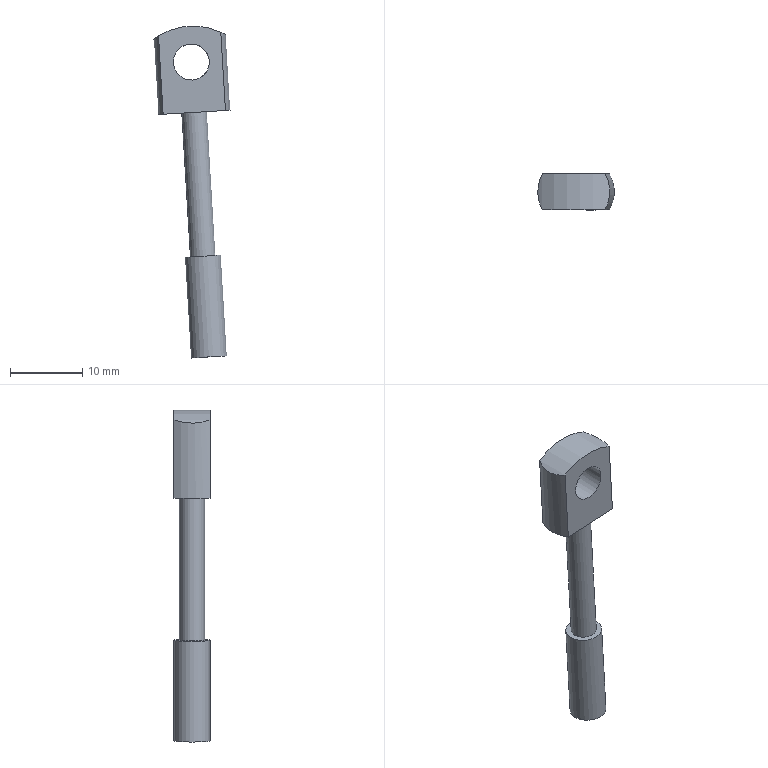Component | NX | PISTON_CONN_ROD | 1 solid | 11 faces | box 10.61 x 5 x 46.08 mm | volume 922 mm3 | cylinder 6 | plane 5 | commonest cylinder face diameters 5 x2 10 x2 18 x1 3.5 x1
STEP:
#1=CARTESIAN_POINT('',(0.,0.,0.));
#2=DIRECTION('',(0.,0.,1.));
#3=DIRECTION('',(1.,0.,0.));
#4=AXIS2_PLACEMENT_3D('',#1,#2,#3);
#5=CARTESIAN_POINT('',(4.091,25.5,90.772));
#6=VERTEX_POINT('',#5);
#7=CARTESIAN_POINT('',(4.091,20.5,90.772));
#8=VERTEX_POINT('',#7);
#9=CARTESIAN_POINT('',(4.091,25.5,90.772));
#10=CARTESIAN_POINT('',(4.534,24.755,90.562));
#11=CARTESIAN_POINT('',(4.784,23.892,90.406));
#12=CARTESIAN_POINT('',(4.783,22.106,90.406));
#13=CARTESIAN_POINT('',(4.534,21.245,90.562));
#14=CARTESIAN_POINT('',(4.091,20.5,90.772));
#15=B_SPLINE_CURVE_WITH_KNOTS('',3,(#9,#10,#11,#12,#13,#14),.UNSPECIFIED.,.F.,.F.,(4,2,4),(0.,0.5,1.),.UNSPECIFIED.);
#16=CARTESIAN_POINT('',(0.2383,20.5,82.638));
#17=DIRECTION('',(0.,1.,0.));
#18=DIRECTION('',(-0.05959,0.,0.9982));
#19=AXIS2_PLACEMENT_3D('',#16,#17,#18);
#20=CYLINDRICAL_SURFACE('',#19,9.);
#21=CARTESIAN_POINT('',(0.5019,5.));
#22=CARTESIAN_POINT('',(0.5069,4.932));
#23=CARTESIAN_POINT('',(0.5164,4.795));
#24=CARTESIAN_POINT('',(0.5296,4.583));
#25=CARTESIAN_POINT('',(0.5416,4.367));
#26=CARTESIAN_POINT('',(0.5524,4.146));
#27=CARTESIAN_POINT('',(0.5619,3.92));
#28=CARTESIAN_POINT('',(0.5701,3.691));
#29=CARTESIAN_POINT('',(0.5768,3.458));
#30=CARTESIAN_POINT('',(0.5822,3.222));
#31=CARTESIAN_POINT('',(0.5861,2.983));
#32=CARTESIAN_POINT('',(0.5885,2.742));
#33=CARTESIAN_POINT('',(0.5893,2.499));
#34=CARTESIAN_POINT('',(0.5885,2.256));
#35=CARTESIAN_POINT('',(0.5861,2.015));
#36=CARTESIAN_POINT('',(0.5822,1.777));
#37=CARTESIAN_POINT('',(0.5768,1.541));
#38=CARTESIAN_POINT('',(0.57,1.308));
#39=CARTESIAN_POINT('',(0.5619,1.079));
#40=CARTESIAN_POINT('',(0.5524,0.8538));
#41=CARTESIAN_POINT('',(0.5416,0.6329));
#42=CARTESIAN_POINT('',(0.5296,0.4165));
#43=CARTESIAN_POINT('',(0.5164,0.2051));
#44=CARTESIAN_POINT('',(0.5069,0.06772));
#45=CARTESIAN_POINT('',(0.5019,0.));
#46=B_SPLINE_CURVE_WITH_KNOTS('',3,(#21,#22,#23,#24,#25,#26,#27,#28,#29,#30,#31,#32,#33,#34,#35,#36,#37,#38,#39,#40,#41,#42,#43,#44,#45),.UNSPECIFIED.,.F.,.F.,(4,1,1,1,1,1,1,1,1,1,1,1,1,1,1,1,1,1,1,1,1,1,4),(0.,0.04545,0.09091,0.1364,0.1818,0.2273,0.2727,0.3182,0.3636,0.4091,0.4545,0.5,0.5455,0.5909,0.6364,0.6818,0.7273,0.7727,0.8182,0.8636,0.9091,0.9545,1.),.QUASI_UNIFORM_KNOTS.);
#47=(GEOMETRIC_REPRESENTATION_CONTEXT(2)PARAMETRIC_REPRESENTATION_CONTEXT()REPRESENTATION_CONTEXT('',''));
#48=DEFINITIONAL_REPRESENTATION('',(#46),#47);
#49=PCURVE('',#20,#48);
#50=CARTESIAN_POINT('',(-0.5363,23.,95.615));
#51=DIRECTION('',(0.05959,0.,-0.9982));
#52=DIRECTION('',(0.,1.,0.));
#53=AXIS2_PLACEMENT_3D('',#50,#51,#52);
#54=CYLINDRICAL_SURFACE('',#53,5.);
#55=CARTESIAN_POINT('',(1.047,5.11));
#56=CARTESIAN_POINT('',(1.063,5.132));
#57=CARTESIAN_POINT('',(1.094,5.173));
#58=CARTESIAN_POINT('',(1.141,5.232));
#59=CARTESIAN_POINT('',(1.188,5.287));
#60=CARTESIAN_POINT('',(1.236,5.337));
#61=CARTESIAN_POINT('',(1.283,5.382));
#62=CARTESIAN_POINT('',(1.33,5.422));
#63=CARTESIAN_POINT('',(1.378,5.455));
#64=CARTESIAN_POINT('',(1.426,5.482));
#65=CARTESIAN_POINT('',(1.474,5.502));
#66=CARTESIAN_POINT('',(1.522,5.514));
#67=CARTESIAN_POINT('',(1.571,5.518));
#68=CARTESIAN_POINT('',(1.62,5.514));
#69=CARTESIAN_POINT('',(1.668,5.502));
#70=CARTESIAN_POINT('',(1.716,5.482));
#71=CARTESIAN_POINT('',(1.764,5.455));
#72=CARTESIAN_POINT('',(1.811,5.422));
#73=CARTESIAN_POINT('',(1.859,5.382));
#74=CARTESIAN_POINT('',(1.906,5.337));
#75=CARTESIAN_POINT('',(1.953,5.287));
#76=CARTESIAN_POINT('',(2.,5.232));
#77=CARTESIAN_POINT('',(2.047,5.173));
#78=CARTESIAN_POINT('',(2.079,5.132));
#79=CARTESIAN_POINT('',(2.094,5.11));
#80=B_SPLINE_CURVE_WITH_KNOTS('',3,(#55,#56,#57,#58,#59,#60,#61,#62,#63,#64,#65,#66,#67,#68,#69,#70,#71,#72,#73,#74,#75,#76,#77,#78,#79),.UNSPECIFIED.,.F.,.F.,(4,1,1,1,1,1,1,1,1,1,1,1,1,1,1,1,1,1,1,1,1,1,4),(0.,0.04545,0.09091,0.1364,0.1818,0.2273,0.2727,0.3182,0.3636,0.4091,0.4545,0.5,0.5455,0.5909,0.6364,0.6818,0.7273,0.7727,0.8182,0.8636,0.9091,0.9545,1.),.QUASI_UNIFORM_KNOTS.);
#81=(GEOMETRIC_REPRESENTATION_CONTEXT(2)PARAMETRIC_REPRESENTATION_CONTEXT()REPRESENTATION_CONTEXT('',''));
#82=DEFINITIONAL_REPRESENTATION('',(#80),#81);
#83=PCURVE('',#54,#82);
#84=SURFACE_CURVE('',#15,(#49,#83),.PCURVE_S1.);
#85=EDGE_CURVE('',#6,#8,#84,.T.);
#86=ORIENTED_EDGE('',*,*,#85,.F.);
#87=CARTESIAN_POINT('',(-4.554,25.5,90.256));
#88=VERTEX_POINT('',#87);
#89=CARTESIAN_POINT('',(0.2383,25.5,82.638));
#90=DIRECTION('',(0.,-1.,0.));
#91=DIRECTION('',(0.9982,0.,0.05959));
#92=AXIS2_PLACEMENT_3D('',#89,#90,#91);
#93=CIRCLE('',#92,9.);
#94=CARTESIAN_POINT('',(1.571,5.));
#95=DIRECTION('',(-1.,0.));
#96=VECTOR('',#95,1.);
#97=LINE('',#94,#96);
#98=(GEOMETRIC_REPRESENTATION_CONTEXT(2)PARAMETRIC_REPRESENTATION_CONTEXT()REPRESENTATION_CONTEXT('',''));
#99=DEFINITIONAL_REPRESENTATION('',(#97),#98);
#100=PCURVE('',#20,#99);
#101=CARTESIAN_POINT('',(0.2383,25.5,82.638));
#102=DIRECTION('',(0.,-1.,0.));
#103=DIRECTION('',(0.05959,0.,-0.9982));
#104=AXIS2_PLACEMENT_3D('',#101,#102,#103);
#105=PLANE('',#104);
#106=CARTESIAN_POINT('',(0.,0.));
#107=DIRECTION('',(-0.,1.));
#108=AXIS2_PLACEMENT_2D('',#106,#107);
#109=CIRCLE('',#108,9.);
#110=(GEOMETRIC_REPRESENTATION_CONTEXT(2)PARAMETRIC_REPRESENTATION_CONTEXT()REPRESENTATION_CONTEXT('',''));
#111=DEFINITIONAL_REPRESENTATION('',(#109),#110);
#112=PCURVE('',#105,#111);
#113=SURFACE_CURVE('',#93,(#100,#112),.PCURVE_S1.);
#114=EDGE_CURVE('',#6,#88,#113,.T.);
#115=ORIENTED_EDGE('',*,*,#114,.T.);
#116=CARTESIAN_POINT('',(-4.554,20.5,90.256));
#117=VERTEX_POINT('',#116);
#118=CARTESIAN_POINT('',(-4.554,25.5,90.256));
#119=CARTESIAN_POINT('',(-4.969,24.755,89.994));
#120=CARTESIAN_POINT('',(-5.199,23.892,89.81));
#121=CARTESIAN_POINT('',(-5.198,22.106,89.81));
#122=CARTESIAN_POINT('',(-4.969,21.245,89.994));
#123=CARTESIAN_POINT('',(-4.554,20.5,90.256));
#124=B_SPLINE_CURVE_WITH_KNOTS('',3,(#118,#119,#120,#121,#122,#123),.UNSPECIFIED.,.F.,.F.,(4,2,4),(0.,0.5,1.),.UNSPECIFIED.);
#125=CARTESIAN_POINT('',(-0.5019,5.));
#126=CARTESIAN_POINT('',(-0.5069,4.932));
#127=CARTESIAN_POINT('',(-0.5164,4.795));
#128=CARTESIAN_POINT('',(-0.5296,4.583));
#129=CARTESIAN_POINT('',(-0.5416,4.367));
#130=CARTESIAN_POINT('',(-0.5524,4.146));
#131=CARTESIAN_POINT('',(-0.5619,3.92));
#132=CARTESIAN_POINT('',(-0.5701,3.691));
#133=CARTESIAN_POINT('',(-0.5768,3.458));
#134=CARTESIAN_POINT('',(-0.5822,3.222));
#135=CARTESIAN_POINT('',(-0.5861,2.983));
#136=CARTESIAN_POINT('',(-0.5885,2.742));
#137=CARTESIAN_POINT('',(-0.5893,2.499));
#138=CARTESIAN_POINT('',(-0.5885,2.256));
#139=CARTESIAN_POINT('',(-0.5861,2.015));
#140=CARTESIAN_POINT('',(-0.5822,1.777));
#141=CARTESIAN_POINT('',(-0.5768,1.541));
#142=CARTESIAN_POINT('',(-0.57,1.308));
#143=CARTESIAN_POINT('',(-0.5619,1.079));
#144=CARTESIAN_POINT('',(-0.5524,0.8538));
#145=CARTESIAN_POINT('',(-0.5416,0.6329));
#146=CARTESIAN_POINT('',(-0.5296,0.4165));
#147=CARTESIAN_POINT('',(-0.5164,0.2051));
#148=CARTESIAN_POINT('',(-0.5069,0.06772));
#149=CARTESIAN_POINT('',(-0.5019,0.));
#150=B_SPLINE_CURVE_WITH_KNOTS('',3,(#125,#126,#127,#128,#129,#130,#131,#132,#133,#134,#135,#136,#137,#138,#139,#140,#141,#142,#143,#144,#145,#146,#147,#148,#149),.UNSPECIFIED.,.F.,.F.,(4,1,1,1,1,1,1,1,1,1,1,1,1,1,1,1,1,1,1,1,1,1,4),(0.,0.04545,0.09091,0.1364,0.1818,0.2273,0.2727,0.3182,0.3636,0.4091,0.4545,0.5,0.5455,0.5909,0.6364,0.6818,0.7273,0.7727,0.8182,0.8636,0.9091,0.9545,1.),.QUASI_UNIFORM_KNOTS.);
#151=(GEOMETRIC_REPRESENTATION_CONTEXT(2)PARAMETRIC_REPRESENTATION_CONTEXT()REPRESENTATION_CONTEXT('',''));
#152=DEFINITIONAL_REPRESENTATION('',(#150),#151);
#153=PCURVE('',#20,#152);
#154=CARTESIAN_POINT('',(-0.5363,23.,95.615));
#155=DIRECTION('',(0.05959,0.,-0.9982));
#156=DIRECTION('',(0.,1.,0.));
#157=AXIS2_PLACEMENT_3D('',#154,#155,#156);
#158=CYLINDRICAL_SURFACE('',#157,5.);
#159=CARTESIAN_POINT('',(5.236,5.11));
#160=CARTESIAN_POINT('',(5.22,5.132));
#161=CARTESIAN_POINT('',(5.189,5.173));
#162=CARTESIAN_POINT('',(5.142,5.232));
#163=CARTESIAN_POINT('',(5.095,5.287));
#164=CARTESIAN_POINT('',(5.048,5.337));
#165=CARTESIAN_POINT('',(5.,5.382));
#166=CARTESIAN_POINT('',(4.953,5.422));
#167=CARTESIAN_POINT('',(4.905,5.455));
#168=CARTESIAN_POINT('',(4.857,5.482));
#169=CARTESIAN_POINT('',(4.809,5.502));
#170=CARTESIAN_POINT('',(4.761,5.514));
#171=CARTESIAN_POINT('',(4.712,5.518));
#172=CARTESIAN_POINT('',(4.664,5.514));
#173=CARTESIAN_POINT('',(4.615,5.502));
#174=CARTESIAN_POINT('',(4.567,5.482));
#175=CARTESIAN_POINT('',(4.519,5.455));
#176=CARTESIAN_POINT('',(4.472,5.422));
#177=CARTESIAN_POINT('',(4.424,5.382));
#178=CARTESIAN_POINT('',(4.377,5.337));
#179=CARTESIAN_POINT('',(4.33,5.287));
#180=CARTESIAN_POINT('',(4.283,5.232));
#181=CARTESIAN_POINT('',(4.236,5.173));
#182=CARTESIAN_POINT('',(4.204,5.132));
#183=CARTESIAN_POINT('',(4.189,5.11));
#184=B_SPLINE_CURVE_WITH_KNOTS('',3,(#159,#160,#161,#162,#163,#164,#165,#166,#167,#168,#169,#170,#171,#172,#173,#174,#175,#176,#177,#178,#179,#180,#181,#182,#183),.UNSPECIFIED.,.F.,.F.,(4,1,1,1,1,1,1,1,1,1,1,1,1,1,1,1,1,1,1,1,1,1,4),(0.,0.04545,0.09091,0.1364,0.1818,0.2273,0.2727,0.3182,0.3636,0.4091,0.4545,0.5,0.5455,0.5909,0.6364,0.6818,0.7273,0.7727,0.8182,0.8636,0.9091,0.9545,1.),.QUASI_UNIFORM_KNOTS.);
#185=(GEOMETRIC_REPRESENTATION_CONTEXT(2)PARAMETRIC_REPRESENTATION_CONTEXT()REPRESENTATION_CONTEXT('',''));
#186=DEFINITIONAL_REPRESENTATION('',(#184),#185);
#187=PCURVE('',#158,#186);
#188=SURFACE_CURVE('',#124,(#153,#187),.PCURVE_S1.);
#189=EDGE_CURVE('',#88,#117,#188,.T.);
#190=ORIENTED_EDGE('',*,*,#189,.T.);
#191=CARTESIAN_POINT('',(0.2383,20.5,82.638));
#192=DIRECTION('',(0.,-1.,0.));
#193=DIRECTION('',(0.9982,0.,0.05959));
#194=AXIS2_PLACEMENT_3D('',#191,#192,#193);
#195=CIRCLE('',#194,9.);
#196=CARTESIAN_POINT('',(1.571,0.));
#197=DIRECTION('',(-1.,0.));
#198=VECTOR('',#197,1.);
#199=LINE('',#196,#198);
#200=(GEOMETRIC_REPRESENTATION_CONTEXT(2)PARAMETRIC_REPRESENTATION_CONTEXT()REPRESENTATION_CONTEXT('',''));
#201=DEFINITIONAL_REPRESENTATION('',(#199),#200);
#202=PCURVE('',#20,#201);
#203=CARTESIAN_POINT('',(0.2383,20.5,82.638));
#204=DIRECTION('',(0.,-1.,0.));
#205=DIRECTION('',(0.05959,0.,-0.9982));
#206=AXIS2_PLACEMENT_3D('',#203,#204,#205);
#207=PLANE('',#206);
#208=CARTESIAN_POINT('',(0.,0.));
#209=DIRECTION('',(-0.,1.));
#210=AXIS2_PLACEMENT_2D('',#208,#209);
#211=CIRCLE('',#210,9.);
#212=(GEOMETRIC_REPRESENTATION_CONTEXT(2)PARAMETRIC_REPRESENTATION_CONTEXT()REPRESENTATION_CONTEXT('',''));
#213=DEFINITIONAL_REPRESENTATION('',(#211),#212);
#214=PCURVE('',#207,#213);
#215=SURFACE_CURVE('',#195,(#202,#214),.PCURVE_S1.);
#216=EDGE_CURVE('',#8,#117,#215,.T.);
#217=ORIENTED_EDGE('',*,*,#216,.F.);
#218=EDGE_LOOP('',(#86,#115,#190,#217));
#219=FACE_BOUND('',#218,.T.);
#220=ADVANCED_FACE('',(#219),#20,.T.);
#221=CARTESIAN_POINT('',(0.149,25.5,84.135));
#222=VERTEX_POINT('',#221);
#223=CARTESIAN_POINT('',(-0.,25.5,86.631));
#224=DIRECTION('',(0.,-1.,0.));
#225=DIRECTION('',(0.05959,0.,-0.9982));
#226=AXIS2_PLACEMENT_3D('',#223,#224,#225);
#227=CIRCLE('',#226,2.5);
#228=CARTESIAN_POINT('',(-4.,0.));
#229=DIRECTION('',(1.,0.));
#230=AXIS2_PLACEMENT_2D('',#228,#229);
#231=CIRCLE('',#230,2.5);
#232=(GEOMETRIC_REPRESENTATION_CONTEXT(2)PARAMETRIC_REPRESENTATION_CONTEXT()REPRESENTATION_CONTEXT('',''));
#233=DEFINITIONAL_REPRESENTATION('',(#231),#232);
#234=PCURVE('',#105,#233);
#235=CARTESIAN_POINT('',(-0.,36.5,86.631));
#236=DIRECTION('',(0.,-1.,0.));
#237=DIRECTION('',(0.05959,0.,-0.9982));
#238=AXIS2_PLACEMENT_3D('',#235,#236,#237);
#239=CYLINDRICAL_SURFACE('',#238,2.5);
#240=CARTESIAN_POINT('',(0.,11.));
#241=DIRECTION('',(1.,0.));
#242=VECTOR('',#241,1.);
#243=LINE('',#240,#242);
#244=(GEOMETRIC_REPRESENTATION_CONTEXT(2)PARAMETRIC_REPRESENTATION_CONTEXT()REPRESENTATION_CONTEXT('',''));
#245=DEFINITIONAL_REPRESENTATION('',(#243),#244);
#246=PCURVE('',#239,#245);
#247=SURFACE_CURVE('',#227,(#234,#246),.PCURVE_S1.);
#248=EDGE_CURVE('',#222,#222,#247,.T.);
#249=ORIENTED_EDGE('',*,*,#248,.T.);
#250=EDGE_LOOP('',(#249));
#251=FACE_BOUND('',#250,.T.);
#252=ORIENTED_EDGE('',*,*,#114,.F.);
#253=CARTESIAN_POINT('',(4.74,25.5,79.901));
#254=VERTEX_POINT('',#253);
#255=CARTESIAN_POINT('',(3.786,25.5,95.873));
#256=DIRECTION('',(0.05959,0.,-0.9982));
#257=VECTOR('',#256,1.);
#258=LINE('',#255,#257);
#259=CARTESIAN_POINT('',(-13.,4.33));
#260=DIRECTION('',(1.,0.));
#261=VECTOR('',#260,1.);
#262=LINE('',#259,#261);
#263=(GEOMETRIC_REPRESENTATION_CONTEXT(2)PARAMETRIC_REPRESENTATION_CONTEXT()REPRESENTATION_CONTEXT('',''));
#264=DEFINITIONAL_REPRESENTATION('',(#262),#263);
#265=PCURVE('',#105,#264);
#266=CARTESIAN_POINT('',(1.047,-0.));
#267=DIRECTION('',(0.,1.));
#268=VECTOR('',#267,1.);
#269=LINE('',#266,#268);
#270=(GEOMETRIC_REPRESENTATION_CONTEXT(2)PARAMETRIC_REPRESENTATION_CONTEXT()REPRESENTATION_CONTEXT('',''));
#271=DEFINITIONAL_REPRESENTATION('',(#269),#270);
#272=PCURVE('',#54,#271);
#273=SURFACE_CURVE('',#258,(#265,#272),.PCURVE_S1.);
#274=EDGE_CURVE('',#6,#254,#273,.T.);
#275=ORIENTED_EDGE('',*,*,#274,.T.);
#276=CARTESIAN_POINT('',(-3.905,25.5,79.385));
#277=VERTEX_POINT('',#276);
#278=CARTESIAN_POINT('',(0.4171,25.5,79.643));
#279=DIRECTION('',(0.9982,0.,0.05959));
#280=VECTOR('',#279,1.);
#281=LINE('',#278,#280);
#282=CARTESIAN_POINT('',(3.,-0.));
#283=DIRECTION('',(-0.,1.));
#284=VECTOR('',#283,1.);
#285=LINE('',#282,#284);
#286=(GEOMETRIC_REPRESENTATION_CONTEXT(2)PARAMETRIC_REPRESENTATION_CONTEXT()REPRESENTATION_CONTEXT('',''));
#287=DEFINITIONAL_REPRESENTATION('',(#285),#286);
#288=PCURVE('',#105,#287);
#289=CARTESIAN_POINT('',(0.4171,20.5,79.643));
#290=DIRECTION('',(-0.05959,0.,0.9982));
#291=DIRECTION('',(0.,-1.,0.));
#292=AXIS2_PLACEMENT_3D('',#289,#290,#291);
#293=PLANE('',#292);
#294=CARTESIAN_POINT('',(-5.,0.));
#295=DIRECTION('',(0.,1.));
#296=VECTOR('',#295,1.);
#297=LINE('',#294,#296);
#298=(GEOMETRIC_REPRESENTATION_CONTEXT(2)PARAMETRIC_REPRESENTATION_CONTEXT()REPRESENTATION_CONTEXT('',''));
#299=DEFINITIONAL_REPRESENTATION('',(#297),#298);
#300=PCURVE('',#293,#299);
#301=SURFACE_CURVE('',#281,(#288,#300),.PCURVE_S1.);
#302=EDGE_CURVE('',#277,#254,#301,.T.);
#303=ORIENTED_EDGE('',*,*,#302,.F.);
#304=CARTESIAN_POINT('',(-4.859,25.5,95.357));
#305=DIRECTION('',(0.05959,0.,-0.9982));
#306=VECTOR('',#305,1.);
#307=LINE('',#304,#306);
#308=CARTESIAN_POINT('',(-13.,-4.33));
#309=DIRECTION('',(1.,0.));
#310=VECTOR('',#309,1.);
#311=LINE('',#308,#310);
#312=(GEOMETRIC_REPRESENTATION_CONTEXT(2)PARAMETRIC_REPRESENTATION_CONTEXT()REPRESENTATION_CONTEXT('',''));
#313=DEFINITIONAL_REPRESENTATION('',(#311),#312);
#314=PCURVE('',#105,#313);
#315=CARTESIAN_POINT('',(5.236,-0.));
#316=DIRECTION('',(0.,1.));
#317=VECTOR('',#316,1.);
#318=LINE('',#315,#317);
#319=(GEOMETRIC_REPRESENTATION_CONTEXT(2)PARAMETRIC_REPRESENTATION_CONTEXT()REPRESENTATION_CONTEXT('',''));
#320=DEFINITIONAL_REPRESENTATION('',(#318),#319);
#321=PCURVE('',#158,#320);
#322=SURFACE_CURVE('',#307,(#314,#321),.PCURVE_S1.);
#323=EDGE_CURVE('',#88,#277,#322,.T.);
#324=ORIENTED_EDGE('',*,*,#323,.F.);
#325=EDGE_LOOP('',(#252,#275,#303,#324));
#326=FACE_BOUND('',#325,.T.);
#327=ADVANCED_FACE('',(#251,#326),#105,.F.);
#328=CARTESIAN_POINT('',(2.496,20.5,86.78));
#329=VERTEX_POINT('',#328);
#330=CARTESIAN_POINT('',(0.149,20.5,84.135));
#331=VERTEX_POINT('',#330);
#332=CARTESIAN_POINT('',(-0.,20.5,86.631));
#333=DIRECTION('',(0.,-1.,0.));
#334=DIRECTION('',(0.9982,0.,0.05959));
#335=AXIS2_PLACEMENT_3D('',#332,#333,#334);
#336=CIRCLE('',#335,2.5);
#337=CARTESIAN_POINT('',(-4.,0.));
#338=DIRECTION('',(0.,1.));
#339=AXIS2_PLACEMENT_2D('',#337,#338);
#340=CIRCLE('',#339,2.5);
#341=(GEOMETRIC_REPRESENTATION_CONTEXT(2)PARAMETRIC_REPRESENTATION_CONTEXT()REPRESENTATION_CONTEXT('',''));
#342=DEFINITIONAL_REPRESENTATION('',(#340),#341);
#343=PCURVE('',#207,#342);
#344=CARTESIAN_POINT('',(1.571,16.));
#345=DIRECTION('',(1.,0.));
#346=VECTOR('',#345,1.);
#347=LINE('',#344,#346);
#348=(GEOMETRIC_REPRESENTATION_CONTEXT(2)PARAMETRIC_REPRESENTATION_CONTEXT()REPRESENTATION_CONTEXT('',''));
#349=DEFINITIONAL_REPRESENTATION('',(#347),#348);
#350=PCURVE('',#239,#349);
#351=SURFACE_CURVE('',#336,(#343,#350),.PCURVE_S1.);
#352=EDGE_CURVE('',#329,#331,#351,.T.);
#353=ORIENTED_EDGE('',*,*,#352,.F.);
#354=CARTESIAN_POINT('',(-0.,20.5,86.631));
#355=DIRECTION('',(0.,-1.,0.));
#356=DIRECTION('',(0.9982,0.,0.05959));
#357=AXIS2_PLACEMENT_3D('',#354,#355,#356);
#358=CIRCLE('',#357,2.5);
#359=CARTESIAN_POINT('',(-4.,0.));
#360=DIRECTION('',(0.,1.));
#361=AXIS2_PLACEMENT_2D('',#359,#360);
#362=CIRCLE('',#361,2.5);
#363=(GEOMETRIC_REPRESENTATION_CONTEXT(2)PARAMETRIC_REPRESENTATION_CONTEXT()REPRESENTATION_CONTEXT('',''));
#364=DEFINITIONAL_REPRESENTATION('',(#362),#363);
#365=PCURVE('',#207,#364);
#366=CARTESIAN_POINT('',(-4.712,16.));
#367=DIRECTION('',(1.,0.));
#368=VECTOR('',#367,1.);
#369=LINE('',#366,#368);
#370=(GEOMETRIC_REPRESENTATION_CONTEXT(2)PARAMETRIC_REPRESENTATION_CONTEXT()REPRESENTATION_CONTEXT('',''));
#371=DEFINITIONAL_REPRESENTATION('',(#369),#370);
#372=PCURVE('',#239,#371);
#373=SURFACE_CURVE('',#358,(#365,#372),.PCURVE_S1.);
#374=EDGE_CURVE('',#331,#329,#373,.T.);
#375=ORIENTED_EDGE('',*,*,#374,.F.);
#376=EDGE_LOOP('',(#353,#375));
#377=FACE_BOUND('',#376,.T.);
#378=CARTESIAN_POINT('',(4.74,20.5,79.901));
#379=VERTEX_POINT('',#378);
#380=CARTESIAN_POINT('',(3.786,20.5,95.873));
#381=DIRECTION('',(0.05959,0.,-0.9982));
#382=VECTOR('',#381,1.);
#383=LINE('',#380,#382);
#384=CARTESIAN_POINT('',(-13.,4.33));
#385=DIRECTION('',(1.,0.));
#386=VECTOR('',#385,1.);
#387=LINE('',#384,#386);
#388=(GEOMETRIC_REPRESENTATION_CONTEXT(2)PARAMETRIC_REPRESENTATION_CONTEXT()REPRESENTATION_CONTEXT('',''));
#389=DEFINITIONAL_REPRESENTATION('',(#387),#388);
#390=PCURVE('',#207,#389);
#391=CARTESIAN_POINT('',(2.094,-0.));
#392=DIRECTION('',(0.,1.));
#393=VECTOR('',#392,1.);
#394=LINE('',#391,#393);
#395=(GEOMETRIC_REPRESENTATION_CONTEXT(2)PARAMETRIC_REPRESENTATION_CONTEXT()REPRESENTATION_CONTEXT('',''));
#396=DEFINITIONAL_REPRESENTATION('',(#394),#395);
#397=PCURVE('',#54,#396);
#398=SURFACE_CURVE('',#383,(#390,#397),.PCURVE_S1.);
#399=EDGE_CURVE('',#8,#379,#398,.T.);
#400=ORIENTED_EDGE('',*,*,#399,.F.);
#401=ORIENTED_EDGE('',*,*,#216,.T.);
#402=CARTESIAN_POINT('',(-3.905,20.5,79.385));
#403=VERTEX_POINT('',#402);
#404=CARTESIAN_POINT('',(-4.859,20.5,95.357));
#405=DIRECTION('',(0.05959,0.,-0.9982));
#406=VECTOR('',#405,1.);
#407=LINE('',#404,#406);
#408=CARTESIAN_POINT('',(-13.,-4.33));
#409=DIRECTION('',(1.,0.));
#410=VECTOR('',#409,1.);
#411=LINE('',#408,#410);
#412=(GEOMETRIC_REPRESENTATION_CONTEXT(2)PARAMETRIC_REPRESENTATION_CONTEXT()REPRESENTATION_CONTEXT('',''));
#413=DEFINITIONAL_REPRESENTATION('',(#411),#412);
#414=PCURVE('',#207,#413);
#415=CARTESIAN_POINT('',(4.189,-0.));
#416=DIRECTION('',(0.,1.));
#417=VECTOR('',#416,1.);
#418=LINE('',#415,#417);
#419=(GEOMETRIC_REPRESENTATION_CONTEXT(2)PARAMETRIC_REPRESENTATION_CONTEXT()REPRESENTATION_CONTEXT('',''));
#420=DEFINITIONAL_REPRESENTATION('',(#418),#419);
#421=PCURVE('',#158,#420);
#422=SURFACE_CURVE('',#407,(#414,#421),.PCURVE_S1.);
#423=EDGE_CURVE('',#117,#403,#422,.T.);
#424=ORIENTED_EDGE('',*,*,#423,.T.);
#425=CARTESIAN_POINT('',(-4.574,20.5,79.345));
#426=DIRECTION('',(0.9982,0.,0.05959));
#427=VECTOR('',#426,1.);
#428=LINE('',#425,#427);
#429=CARTESIAN_POINT('',(3.,-5.));
#430=DIRECTION('',(-0.,1.));
#431=VECTOR('',#430,1.);
#432=LINE('',#429,#431);
#433=(GEOMETRIC_REPRESENTATION_CONTEXT(2)PARAMETRIC_REPRESENTATION_CONTEXT()REPRESENTATION_CONTEXT('',''));
#434=DEFINITIONAL_REPRESENTATION('',(#432),#433);
#435=PCURVE('',#207,#434);
#436=CARTESIAN_POINT('',(0.,-5.));
#437=DIRECTION('',(0.,1.));
#438=VECTOR('',#437,1.);
#439=LINE('',#436,#438);
#440=(GEOMETRIC_REPRESENTATION_CONTEXT(2)PARAMETRIC_REPRESENTATION_CONTEXT()REPRESENTATION_CONTEXT('',''));
#441=DEFINITIONAL_REPRESENTATION('',(#439),#440);
#442=PCURVE('',#293,#441);
#443=SURFACE_CURVE('',#428,(#435,#442),.PCURVE_S1.);
#444=EDGE_CURVE('',#403,#379,#443,.T.);
#445=ORIENTED_EDGE('',*,*,#444,.T.);
#446=EDGE_LOOP('',(#400,#401,#424,#445));
#447=FACE_BOUND('',#446,.T.);
#448=ADVANCED_FACE('',(#377,#447),#207,.T.);
#449=CARTESIAN_POINT('',(1.609,21.25,59.679));
#450=VERTEX_POINT('',#449);
#451=CARTESIAN_POINT('',(1.609,23.,59.679));
#452=DIRECTION('',(-0.05959,0.,0.9982));
#453=DIRECTION('',(0.,-1.,0.));
#454=AXIS2_PLACEMENT_3D('',#451,#452,#453);
#455=CIRCLE('',#454,1.75);
#456=CARTESIAN_POINT('',(1.609,23.,59.679));
#457=DIRECTION('',(-0.05959,0.,0.9982));
#458=DIRECTION('',(0.,-1.,0.));
#459=AXIS2_PLACEMENT_3D('',#456,#457,#458);
#460=PLANE('',#459);
#461=CARTESIAN_POINT('',(0.,0.));
#462=DIRECTION('',(1.,0.));
#463=AXIS2_PLACEMENT_2D('',#461,#462);
#464=CIRCLE('',#463,1.75);
#465=(GEOMETRIC_REPRESENTATION_CONTEXT(2)PARAMETRIC_REPRESENTATION_CONTEXT()REPRESENTATION_CONTEXT('',''));
#466=DEFINITIONAL_REPRESENTATION('',(#464),#465);
#467=PCURVE('',#460,#466);
#468=CARTESIAN_POINT('',(1.609,23.,59.679));
#469=DIRECTION('',(-0.05959,0.,0.9982));
#470=DIRECTION('',(0.,-1.,0.));
#471=AXIS2_PLACEMENT_3D('',#468,#469,#470);
#472=CYLINDRICAL_SURFACE('',#471,1.75);
#473=CARTESIAN_POINT('',(0.,0.));
#474=DIRECTION('',(1.,0.));
#475=VECTOR('',#474,1.);
#476=LINE('',#473,#475);
#477=(GEOMETRIC_REPRESENTATION_CONTEXT(2)PARAMETRIC_REPRESENTATION_CONTEXT()REPRESENTATION_CONTEXT('',''));
#478=DEFINITIONAL_REPRESENTATION('',(#476),#477);
#479=PCURVE('',#472,#478);
#480=SURFACE_CURVE('',#455,(#467,#479),.PCURVE_S1.);
#481=EDGE_CURVE('',#450,#450,#480,.T.);
#482=ORIENTED_EDGE('',*,*,#481,.F.);
#483=EDGE_LOOP('',(#482));
#484=FACE_BOUND('',#483,.T.);
#485=CARTESIAN_POINT('',(1.609,20.5,59.679));
#486=VERTEX_POINT('',#485);
#487=CARTESIAN_POINT('',(1.609,23.,59.679));
#488=DIRECTION('',(0.05959,0.,-0.9982));
#489=DIRECTION('',(0.,-1.,0.));
#490=AXIS2_PLACEMENT_3D('',#487,#488,#489);
#491=CIRCLE('',#490,2.5);
#492=CARTESIAN_POINT('',(2.5,0.));
#493=CARTESIAN_POINT('',(2.5,-4.33));
#494=CARTESIAN_POINT('',(-1.25,-2.165));
#495=CARTESIAN_POINT('',(-5.,-0.));
#496=CARTESIAN_POINT('',(-1.25,2.165));
#497=CARTESIAN_POINT('',(2.5,4.33));
#498=CARTESIAN_POINT('',(2.5,0.));
#499=(BOUNDED_CURVE()B_SPLINE_CURVE(2,(#492,#493,#494,#495,#496,#497,#498),.UNSPECIFIED.,.T.,.F.)B_SPLINE_CURVE_WITH_KNOTS((1,2,2,2,2,1),(-2.094,0.,2.094,4.189,6.283,8.378),.UNSPECIFIED.)CURVE()GEOMETRIC_REPRESENTATION_ITEM()RATIONAL_B_SPLINE_CURVE((1.,0.5,1.,0.5,1.,0.5,1.))REPRESENTATION_ITEM(''));
#500=(GEOMETRIC_REPRESENTATION_CONTEXT(2)PARAMETRIC_REPRESENTATION_CONTEXT()REPRESENTATION_CONTEXT('',''));
#501=DEFINITIONAL_REPRESENTATION('',(#499),#500);
#502=PCURVE('',#460,#501);
#503=CARTESIAN_POINT('',(2.443,23.,45.704));
#504=DIRECTION('',(-0.05959,0.,0.9982));
#505=DIRECTION('',(0.,-1.,0.));
#506=AXIS2_PLACEMENT_3D('',#503,#504,#505);
#507=CYLINDRICAL_SURFACE('',#506,2.5);
#508=CARTESIAN_POINT('',(6.283,14.));
#509=DIRECTION('',(-1.,0.));
#510=VECTOR('',#509,1.);
#511=LINE('',#508,#510);
#512=(GEOMETRIC_REPRESENTATION_CONTEXT(2)PARAMETRIC_REPRESENTATION_CONTEXT()REPRESENTATION_CONTEXT('',''));
#513=DEFINITIONAL_REPRESENTATION('',(#511),#512);
#514=PCURVE('',#507,#513);
#515=SURFACE_CURVE('',#491,(#502,#514),.PCURVE_S1.);
#516=EDGE_CURVE('',#486,#486,#515,.T.);
#517=ORIENTED_EDGE('',*,*,#516,.F.);
#518=EDGE_LOOP('',(#517));
#519=FACE_BOUND('',#518,.T.);
#520=ADVANCED_FACE('',(#484,#519),#460,.T.);
#521=CARTESIAN_POINT('',(2.443,20.5,45.704));
#522=VERTEX_POINT('',#521);
#523=CARTESIAN_POINT('',(2.443,23.,45.704));
#524=DIRECTION('',(-0.05959,0.,0.9982));
#525=DIRECTION('',(0.,-1.,0.));
#526=AXIS2_PLACEMENT_3D('',#523,#524,#525);
#527=CIRCLE('',#526,2.5);
#528=CARTESIAN_POINT('',(2.443,23.,45.704));
#529=DIRECTION('',(0.05959,0.,-0.9982));
#530=DIRECTION('',(0.,1.,0.));
#531=AXIS2_PLACEMENT_3D('',#528,#529,#530);
#532=PLANE('',#531);
#533=CARTESIAN_POINT('',(-2.5,0.));
#534=CARTESIAN_POINT('',(-2.5,4.33));
#535=CARTESIAN_POINT('',(1.25,2.165));
#536=CARTESIAN_POINT('',(5.,0.));
#537=CARTESIAN_POINT('',(1.25,-2.165));
#538=CARTESIAN_POINT('',(-2.5,-4.33));
#539=CARTESIAN_POINT('',(-2.5,0.));
#540=(BOUNDED_CURVE()B_SPLINE_CURVE(2,(#533,#534,#535,#536,#537,#538,#539),.UNSPECIFIED.,.T.,.F.)B_SPLINE_CURVE_WITH_KNOTS((1,2,2,2,2,1),(-2.094,0.,2.094,4.189,6.283,8.378),.UNSPECIFIED.)CURVE()GEOMETRIC_REPRESENTATION_ITEM()RATIONAL_B_SPLINE_CURVE((1.,0.5,1.,0.5,1.,0.5,1.))REPRESENTATION_ITEM(''));
#541=(GEOMETRIC_REPRESENTATION_CONTEXT(2)PARAMETRIC_REPRESENTATION_CONTEXT()REPRESENTATION_CONTEXT('',''));
#542=DEFINITIONAL_REPRESENTATION('',(#540),#541);
#543=PCURVE('',#532,#542);
#544=CARTESIAN_POINT('',(0.,0.));
#545=DIRECTION('',(1.,0.));
#546=VECTOR('',#545,1.);
#547=LINE('',#544,#546);
#548=(GEOMETRIC_REPRESENTATION_CONTEXT(2)PARAMETRIC_REPRESENTATION_CONTEXT()REPRESENTATION_CONTEXT('',''));
#549=DEFINITIONAL_REPRESENTATION('',(#547),#548);
#550=PCURVE('',#507,#549);
#551=SURFACE_CURVE('',#527,(#543,#550),.PCURVE_S1.);
#552=EDGE_CURVE('',#522,#522,#551,.T.);
#553=ORIENTED_EDGE('',*,*,#552,.F.);
#554=EDGE_LOOP('',(#553));
#555=FACE_BOUND('',#554,.T.);
#556=ADVANCED_FACE('',(#555),#532,.T.);
#557=ORIENTED_EDGE('',*,*,#516,.T.);
#558=CARTESIAN_POINT('',(2.443,20.5,45.704));
#559=CARTESIAN_POINT('',(1.609,20.5,59.679));
#560=B_SPLINE_CURVE_WITH_KNOTS('',1,(#558,#559),.UNSPECIFIED.,.F.,.F.,(2,2),(0.,14.),.PIECEWISE_BEZIER_KNOTS.);
#561=CARTESIAN_POINT('',(0.,0.));
#562=DIRECTION('',(0.,1.));
#563=VECTOR('',#562,1.);
#564=LINE('',#561,#563);
#565=(GEOMETRIC_REPRESENTATION_CONTEXT(2)PARAMETRIC_REPRESENTATION_CONTEXT()REPRESENTATION_CONTEXT('',''));
#566=DEFINITIONAL_REPRESENTATION('',(#564),#565);
#567=PCURVE('',#507,#566);
#568=CARTESIAN_POINT('',(6.283,0.));
#569=DIRECTION('',(0.,1.));
#570=VECTOR('',#569,1.);
#571=LINE('',#568,#570);
#572=(GEOMETRIC_REPRESENTATION_CONTEXT(2)PARAMETRIC_REPRESENTATION_CONTEXT()REPRESENTATION_CONTEXT('',''));
#573=DEFINITIONAL_REPRESENTATION('',(#571),#572);
#574=PCURVE('',#507,#573);
#575=SEAM_CURVE('',#560,(#567,#574),.PCURVE_S1.);
#576=EDGE_CURVE('',#522,#486,#575,.T.);
#577=ORIENTED_EDGE('',*,*,#576,.F.);
#578=ORIENTED_EDGE('',*,*,#552,.T.);
#579=ORIENTED_EDGE('',*,*,#576,.T.);
#580=EDGE_LOOP('',(#557,#577,#578,#579));
#581=FACE_BOUND('',#580,.T.);
#582=ADVANCED_FACE('',(#581),#507,.T.);
#583=CARTESIAN_POINT('',(0.4171,21.25,79.643));
#584=VERTEX_POINT('',#583);
#585=CARTESIAN_POINT('',(0.4171,23.,79.643));
#586=DIRECTION('',(-0.05959,0.,0.9982));
#587=DIRECTION('',(0.,-1.,0.));
#588=AXIS2_PLACEMENT_3D('',#585,#586,#587);
#589=CIRCLE('',#588,1.75);
#590=CARTESIAN_POINT('',(0.,20.));
#591=DIRECTION('',(1.,0.));
#592=VECTOR('',#591,1.);
#593=LINE('',#590,#592);
#594=(GEOMETRIC_REPRESENTATION_CONTEXT(2)PARAMETRIC_REPRESENTATION_CONTEXT()REPRESENTATION_CONTEXT('',''));
#595=DEFINITIONAL_REPRESENTATION('',(#593),#594);
#596=PCURVE('',#472,#595);
#597=CARTESIAN_POINT('',(-2.5,0.));
#598=DIRECTION('',(1.,0.));
#599=AXIS2_PLACEMENT_2D('',#597,#598);
#600=CIRCLE('',#599,1.75);
#601=(GEOMETRIC_REPRESENTATION_CONTEXT(2)PARAMETRIC_REPRESENTATION_CONTEXT()REPRESENTATION_CONTEXT('',''));
#602=DEFINITIONAL_REPRESENTATION('',(#600),#601);
#603=PCURVE('',#293,#602);
#604=SURFACE_CURVE('',#589,(#596,#603),.PCURVE_S1.);
#605=EDGE_CURVE('',#584,#584,#604,.T.);
#606=ORIENTED_EDGE('',*,*,#605,.F.);
#607=CARTESIAN_POINT('',(1.609,21.25,59.679));
#608=CARTESIAN_POINT('',(0.4171,21.25,79.643));
#609=B_SPLINE_CURVE_WITH_KNOTS('',1,(#607,#608),.UNSPECIFIED.,.F.,.F.,(2,2),(0.,20.),.PIECEWISE_BEZIER_KNOTS.);
#610=CARTESIAN_POINT('',(0.,0.));
#611=DIRECTION('',(0.,1.));
#612=VECTOR('',#611,1.);
#613=LINE('',#610,#612);
#614=(GEOMETRIC_REPRESENTATION_CONTEXT(2)PARAMETRIC_REPRESENTATION_CONTEXT()REPRESENTATION_CONTEXT('',''));
#615=DEFINITIONAL_REPRESENTATION('',(#613),#614);
#616=PCURVE('',#472,#615);
#617=CARTESIAN_POINT('',(6.283,0.));
#618=DIRECTION('',(0.,1.));
#619=VECTOR('',#618,1.);
#620=LINE('',#617,#619);
#621=(GEOMETRIC_REPRESENTATION_CONTEXT(2)PARAMETRIC_REPRESENTATION_CONTEXT()REPRESENTATION_CONTEXT('',''));
#622=DEFINITIONAL_REPRESENTATION('',(#620),#621);
#623=PCURVE('',#472,#622);
#624=SEAM_CURVE('',#609,(#616,#623),.PCURVE_S1.);
#625=EDGE_CURVE('',#450,#584,#624,.T.);
#626=ORIENTED_EDGE('',*,*,#625,.F.);
#627=ORIENTED_EDGE('',*,*,#481,.T.);
#628=ORIENTED_EDGE('',*,*,#625,.T.);
#629=EDGE_LOOP('',(#606,#626,#627,#628));
#630=FACE_BOUND('',#629,.T.);
#631=ADVANCED_FACE('',(#630),#472,.T.);
#632=ORIENTED_EDGE('',*,*,#302,.T.);
#633=CARTESIAN_POINT('',(0.4171,23.,79.643));
#634=DIRECTION('',(0.05959,0.,-0.9982));
#635=DIRECTION('',(-0.9982,0.,-0.05959));
#636=AXIS2_PLACEMENT_3D('',#633,#634,#635);
#637=CIRCLE('',#636,5.);
#638=CARTESIAN_POINT('',(-2.5,-5.));
#639=CARTESIAN_POINT('',(-11.16,-5.));
#640=CARTESIAN_POINT('',(-6.83,2.5));
#641=CARTESIAN_POINT('',(-2.5,10.));
#642=CARTESIAN_POINT('',(1.83,2.5));
#643=CARTESIAN_POINT('',(6.16,-5.));
#644=CARTESIAN_POINT('',(-2.5,-5.));
#645=(BOUNDED_CURVE()B_SPLINE_CURVE(2,(#638,#639,#640,#641,#642,#643,#644),.UNSPECIFIED.,.T.,.F.)B_SPLINE_CURVE_WITH_KNOTS((1,2,2,2,2,1),(-2.094,0.,2.094,4.189,6.283,8.378),.UNSPECIFIED.)CURVE()GEOMETRIC_REPRESENTATION_ITEM()RATIONAL_B_SPLINE_CURVE((1.,0.5,1.,0.5,1.,0.5,1.))REPRESENTATION_ITEM(''));
#646=(GEOMETRIC_REPRESENTATION_CONTEXT(2)PARAMETRIC_REPRESENTATION_CONTEXT()REPRESENTATION_CONTEXT('',''));
#647=DEFINITIONAL_REPRESENTATION('',(#645),#646);
#648=PCURVE('',#293,#647);
#649=CARTESIAN_POINT('',(-1.571,16.));
#650=DIRECTION('',(1.,0.));
#651=VECTOR('',#650,1.);
#652=LINE('',#649,#651);
#653=(GEOMETRIC_REPRESENTATION_CONTEXT(2)PARAMETRIC_REPRESENTATION_CONTEXT()REPRESENTATION_CONTEXT('',''));
#654=DEFINITIONAL_REPRESENTATION('',(#652),#653);
#655=PCURVE('',#54,#654);
#656=SURFACE_CURVE('',#637,(#648,#655),.PCURVE_S1.);
#657=EDGE_CURVE('',#254,#379,#656,.T.);
#658=ORIENTED_EDGE('',*,*,#657,.T.);
#659=ORIENTED_EDGE('',*,*,#444,.F.);
#660=CARTESIAN_POINT('',(0.4171,23.,79.643));
#661=DIRECTION('',(-0.05959,0.,0.9982));
#662=DIRECTION('',(0.9982,0.,0.05959));
#663=AXIS2_PLACEMENT_3D('',#660,#661,#662);
#664=CIRCLE('',#663,5.);
#665=CARTESIAN_POINT('',(-2.5,0.));
#666=DIRECTION('',(0.,1.));
#667=AXIS2_PLACEMENT_2D('',#665,#666);
#668=CIRCLE('',#667,5.);
#669=(GEOMETRIC_REPRESENTATION_CONTEXT(2)PARAMETRIC_REPRESENTATION_CONTEXT()REPRESENTATION_CONTEXT('',''));
#670=DEFINITIONAL_REPRESENTATION('',(#668),#669);
#671=PCURVE('',#293,#670);
#672=CARTESIAN_POINT('',(7.854,16.));
#673=DIRECTION('',(-1.,0.));
#674=VECTOR('',#673,1.);
#675=LINE('',#672,#674);
#676=(GEOMETRIC_REPRESENTATION_CONTEXT(2)PARAMETRIC_REPRESENTATION_CONTEXT()REPRESENTATION_CONTEXT('',''));
#677=DEFINITIONAL_REPRESENTATION('',(#675),#676);
#678=PCURVE('',#158,#677);
#679=SURFACE_CURVE('',#664,(#671,#678),.PCURVE_S1.);
#680=EDGE_CURVE('',#277,#403,#679,.T.);
#681=ORIENTED_EDGE('',*,*,#680,.F.);
#682=EDGE_LOOP('',(#632,#658,#659,#681));
#683=FACE_BOUND('',#682,.T.);
#684=ORIENTED_EDGE('',*,*,#605,.T.);
#685=EDGE_LOOP('',(#684));
#686=FACE_BOUND('',#685,.T.);
#687=ADVANCED_FACE('',(#683,#686),#293,.F.);
#688=ORIENTED_EDGE('',*,*,#189,.F.);
#689=ORIENTED_EDGE('',*,*,#323,.T.);
#690=ORIENTED_EDGE('',*,*,#680,.T.);
#691=ORIENTED_EDGE('',*,*,#423,.F.);
#692=EDGE_LOOP('',(#688,#689,#690,#691));
#693=FACE_BOUND('',#692,.T.);
#694=ADVANCED_FACE('',(#693),#158,.T.);
#695=ORIENTED_EDGE('',*,*,#85,.T.);
#696=ORIENTED_EDGE('',*,*,#399,.T.);
#697=ORIENTED_EDGE('',*,*,#657,.F.);
#698=ORIENTED_EDGE('',*,*,#274,.F.);
#699=EDGE_LOOP('',(#695,#696,#697,#698));
#700=FACE_BOUND('',#699,.T.);
#701=ADVANCED_FACE('',(#700),#54,.T.);
#702=ORIENTED_EDGE('',*,*,#374,.F.);
#703=CARTESIAN_POINT('',(0.149,25.5,84.135));
#704=CARTESIAN_POINT('',(0.149,20.5,84.135));
#705=B_SPLINE_CURVE_WITH_KNOTS('',1,(#703,#704),.UNSPECIFIED.,.F.,.F.,(2,2),(11.,16.),.PIECEWISE_BEZIER_KNOTS.);
#706=CARTESIAN_POINT('',(0.,0.));
#707=DIRECTION('',(0.,1.));
#708=VECTOR('',#707,1.);
#709=LINE('',#706,#708);
#710=(GEOMETRIC_REPRESENTATION_CONTEXT(2)PARAMETRIC_REPRESENTATION_CONTEXT()REPRESENTATION_CONTEXT('',''));
#711=DEFINITIONAL_REPRESENTATION('',(#709),#710);
#712=PCURVE('',#239,#711);
#713=CARTESIAN_POINT('',(6.283,0.));
#714=DIRECTION('',(0.,1.));
#715=VECTOR('',#714,1.);
#716=LINE('',#713,#715);
#717=(GEOMETRIC_REPRESENTATION_CONTEXT(2)PARAMETRIC_REPRESENTATION_CONTEXT()REPRESENTATION_CONTEXT('',''));
#718=DEFINITIONAL_REPRESENTATION('',(#716),#717);
#719=PCURVE('',#239,#718);
#720=SEAM_CURVE('',#705,(#712,#719),.PCURVE_S1.);
#721=EDGE_CURVE('',#222,#331,#720,.T.);
#722=ORIENTED_EDGE('',*,*,#721,.F.);
#723=ORIENTED_EDGE('',*,*,#248,.T.);
#724=ORIENTED_EDGE('',*,*,#721,.T.);
#725=ORIENTED_EDGE('',*,*,#352,.F.);
#726=EDGE_LOOP('',(#702,#722,#723,#724,#725));
#727=FACE_BOUND('',#726,.F.);
#728=ADVANCED_FACE('',(#727),#239,.F.);
#729=CLOSED_SHELL('',(#220,#327,#448,#520,#556,#582,#631,#687,#694,#701,#728));
#730=MANIFOLD_SOLID_BREP('',#729);
#731=(LENGTH_UNIT()NAMED_UNIT(*)SI_UNIT(.MILLI.,.METRE.));
#732=UNCERTAINTY_MEASURE_WITH_UNIT(LENGTH_MEASURE(0.0002),#731,'','');
#733=(NAMED_UNIT(*)PLANE_ANGLE_UNIT()SI_UNIT($,.RADIAN.));
#734=(NAMED_UNIT(*)SI_UNIT($,.STERADIAN.)SOLID_ANGLE_UNIT());
#735=(GEOMETRIC_REPRESENTATION_CONTEXT(3)GLOBAL_UNCERTAINTY_ASSIGNED_CONTEXT((#732))GLOBAL_UNIT_ASSIGNED_CONTEXT((#731,#733,#734))REPRESENTATION_CONTEXT('',''));
#736=ADVANCED_BREP_SHAPE_REPRESENTATION('',(#4,#730),#735);